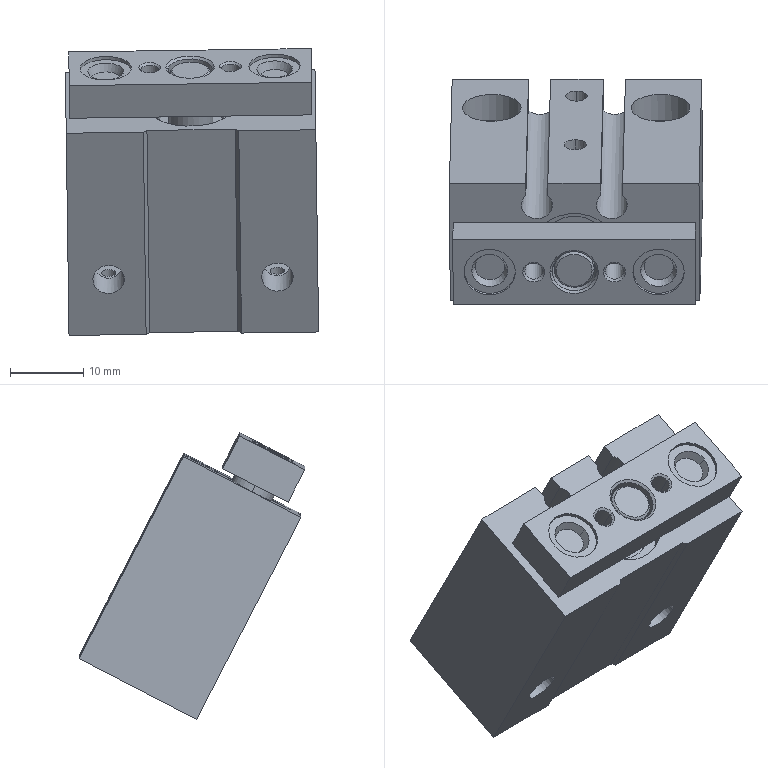Component | SolidWorks | PurchasedPart;Three-axisCylinderTCM10x5S-1 | 2 solids | 142 faces | volume 17545 mm3 | cylinder 70 | plane 48 | cone 24 | commonest cylinder face diameters 6 x14 2.459 x8 3.242 x8 4.3 x8 4.2 x6 7 x4 10 x4 3 x4